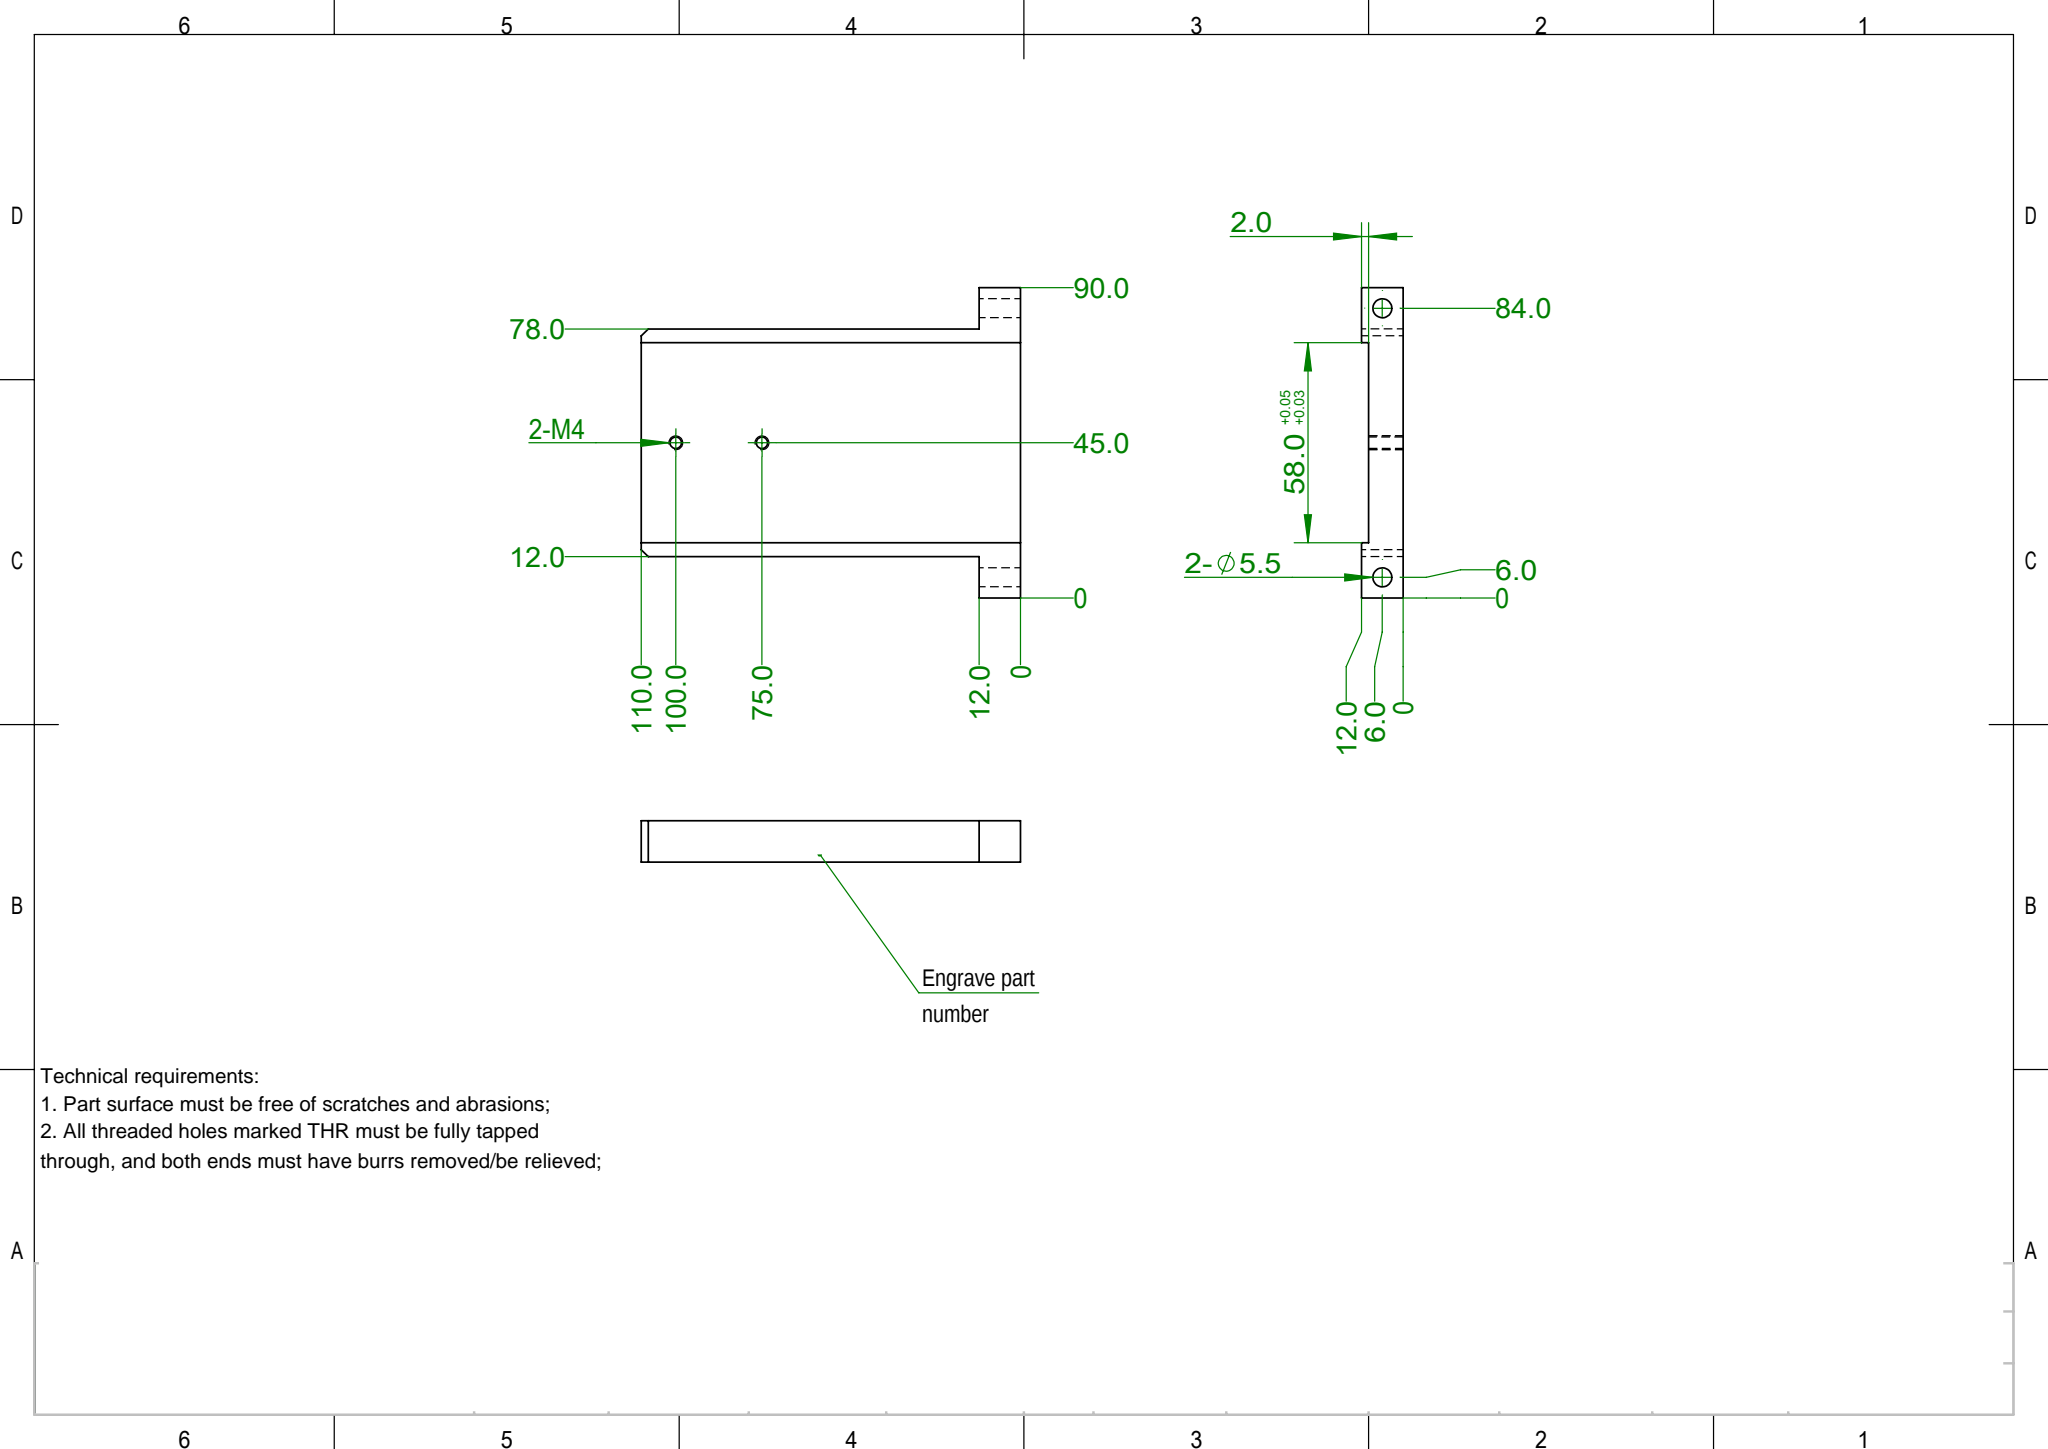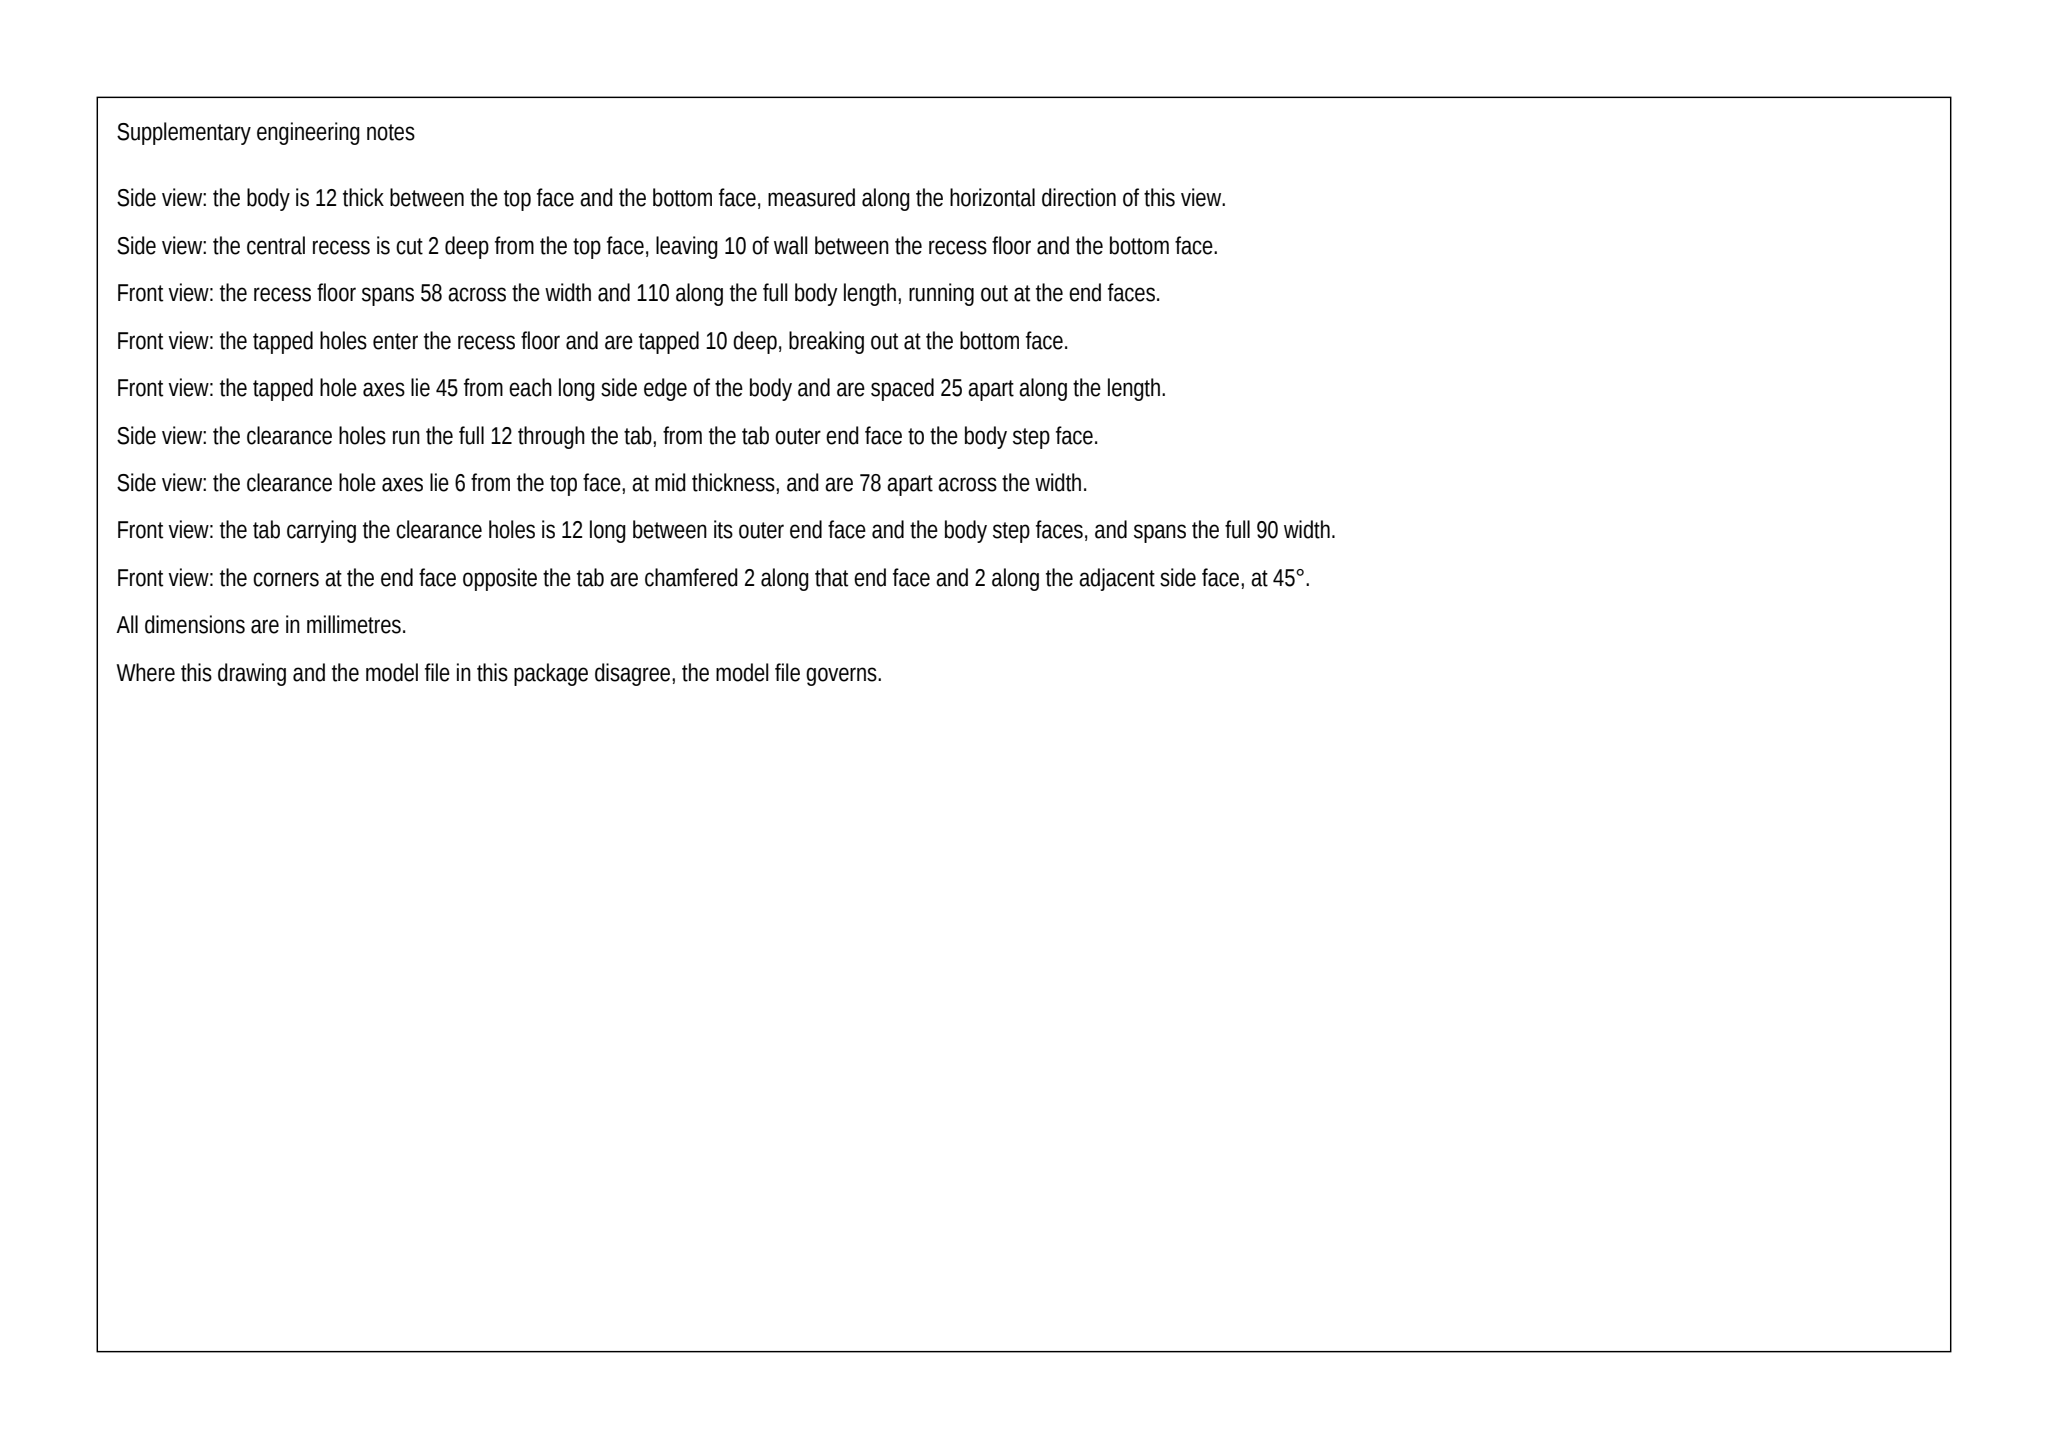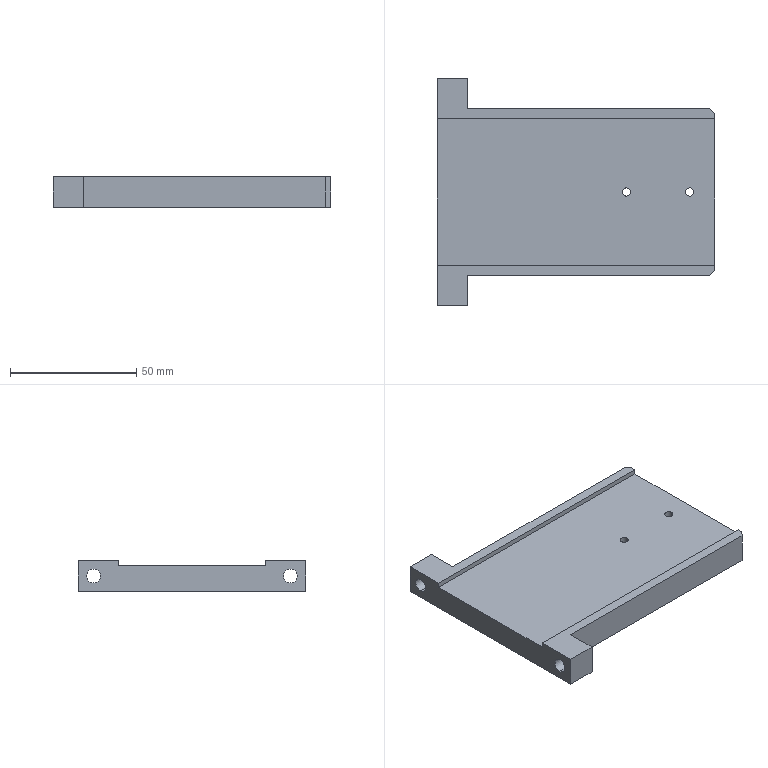Part | SolidWorks | mm | 1 solid | 24 faces | box 110 x 90 x 12 mm | volume 77027 mm3 | plane 16 | cylinder 8 | commonest cylinder face diameters 3.3 x4 5.5 x4
Drawing notes:
FRONT VIEW: 2X C4 ON 110 END CORNERS AT 12.0 & 78.0 | from the solid: y-planes at 16.0 and 74.0 (4 mm in from y=12 and y=78) adjacent to x=110 end face; corner cut 4x4
2.0 DEEP CHANNEL 58.0 WIDE: 16.0 FROM 0 EDGE, SYM ABT 45.0 CL | from the solid: y-planes at 16.0 and 74.0 (58.0 wide) within 0-90 bbox; x-planes 12.0 vs 10.0 give 2.0 depth; midpoint 45.0
2X M4 TAPPED HOLE (Ø3.3 DRILL) 10.0 DEEP, BLIND FROM THE 12.0 TOP FACE (Z=12.0); AT X=75.0 AND X=100.0, Y=45.0 FROM 0 EDGES | from the solid: cylinders [3.3, z, (75.0,45.0), length 10.0] and [3.3, z, (100.0,45.0), length 10.0]; bbox z = 12.0
2.0 DEEP x 58.0 WIDE CHANNEL (Y 16.0 TO 74.0) RUNS FULL LENGTH, X=0 THRU X=110.0; FLOOR AT Z=10.0 | from the solid: axis_planes z=10.0 (channel floor, 1 face) and z=12.0 (top split into 2 faces); single faces at x=0.0 and x=110.0 with bbox x = 110.0; y planes 16.0 and 74.0
build123d program:
from build123d import *

# Parameters (mm, degrees)
SKETCH1_W                  = 105
SKETCH1_H                  = 90
BOSS_EXTRUDE1_DEPTH        = 6
SKETCH2_W                  = 105
SKETCH2_H                  = 58
CUT_EXTRUDE1_DEPTH         = 2
SKETCH3_W                  = 93
SKETCH3_H                  = 12
CUT_EXTRUDE2_DEPTH         = 71.18
F_5_5_5_5_DIAMETER_HOLE1_D = 5.5
M4_TAPPED_HOLE1_D          = 3.3
MOVE_FACE1_BY              = 5
CHAMFER1_SIZE              = 2


with BuildPart() as part:
    # Sketch1 → Boss-Extrude1 (new, symmetric)
    with BuildSketch(Plane.XY):
        Rectangle(SKETCH1_W, SKETCH1_H)
    extrude(amount=BOSS_EXTRUDE1_DEPTH, both=True)

    # Sketch2 → Cut-Extrude1 (cut)
    with BuildSketch(Plane.XY.offset(6)):
        Rectangle(SKETCH2_W, SKETCH2_H)
    extrude(amount=-CUT_EXTRUDE1_DEPTH, mode=Mode.SUBTRACT)

    # Sketch3 → Cut-Extrude2 (cut, through all)
    with BuildSketch(Plane.XY.offset(6)):
        with Locations((6, 39)):
            Rectangle(SKETCH3_W, SKETCH3_H)
        with Locations((6, -39)):
            Rectangle(SKETCH3_W, SKETCH3_H)
    extrude(amount=-CUT_EXTRUDE2_DEPTH, mode=Mode.SUBTRACT)

    # 5.5 _5.5_ Diameter Hole1 (through all)
    with Locations(Plane(origin=(-40.5, 0, 0), x_dir=(0, 0, -1), z_dir=(1, 0, 0))):
        with Locations((0, -39), (0, 39)):
            Hole(F_5_5_5_5_DIAMETER_HOLE1_D / 2)

    # M4 Tapped Hole1 (through all)
    with Locations(Plane.XY.offset(4)):
        with Locations((22.5, 0), (47.5, 0)):
            Hole(M4_TAPPED_HOLE1_D / 2)

    # Move Face1: a face moved outward by 5.0
    extrude(part.faces().sort_by_distance((52.5, 0, -0.858))[0], amount=MOVE_FACE1_BY, dir=(1, 0, 0))

    # Chamfer1
    chamfer1_edges = [part.edges().sort_by_distance(p)[0] for p in [
        (57.5, 33, 0),
        (57.5, -33, 0),
    ]]
    chamfer(chamfer1_edges, length=CHAMFER1_SIZE)


solid = part.part
STEP:
#1=CARTESIAN_POINT('',(20.85,-0.,-6.));
#2=VERTEX_POINT('',#1);
#3=CARTESIAN_POINT('',(24.15,-0.,-6.));
#4=VERTEX_POINT('',#3);
#5=CARTESIAN_POINT('',(22.5,-0.,-6.));
#6=DIRECTION('',(0.,0.,1.));
#7=DIRECTION('',(1.,0.,0.));
#8=AXIS2_PLACEMENT_3D('',#5,#6,#7);
#9=CIRCLE('',#8,1.65);
#10=EDGE_CURVE('',#2,#4,#9,.T.);
#11=ORIENTED_EDGE('',*,*,#10,.F.);
#12=CARTESIAN_POINT('',(20.85,-0.,4.));
#13=VERTEX_POINT('',#12);
#14=CARTESIAN_POINT('',(20.85,-0.,4.));
#15=DIRECTION('',(0.,0.,1.));
#16=VECTOR('',#15,1000.);
#17=LINE('',#14,#16);
#18=EDGE_CURVE('',#2,#13,#17,.T.);
#19=ORIENTED_EDGE('',*,*,#18,.T.);
#20=CARTESIAN_POINT('',(24.15,-0.,4.));
#21=VERTEX_POINT('',#20);
#22=CARTESIAN_POINT('',(22.5,-0.,4.));
#23=DIRECTION('',(0.,0.,1.));
#24=DIRECTION('',(1.,0.,0.));
#25=AXIS2_PLACEMENT_3D('',#22,#23,#24);
#26=CIRCLE('',#25,1.65);
#27=EDGE_CURVE('',#13,#21,#26,.T.);
#28=ORIENTED_EDGE('',*,*,#27,.T.);
#29=CARTESIAN_POINT('',(24.15,-0.,4.));
#30=DIRECTION('',(0.,0.,1.));
#31=VECTOR('',#30,1000.);
#32=LINE('',#29,#31);
#33=EDGE_CURVE('',#4,#21,#32,.T.);
#34=ORIENTED_EDGE('',*,*,#33,.F.);
#35=EDGE_LOOP('',(#11,#19,#28,#34));
#36=FACE_OUTER_BOUND('',#35,.T.);
#37=CARTESIAN_POINT('',(22.5,-0.,4.));
#38=DIRECTION('',(0.,0.,1.));
#39=DIRECTION('',(1.,0.,0.));
#40=AXIS2_PLACEMENT_3D('',#37,#38,#39);
#41=CYLINDRICAL_SURFACE('',#40,1.65);
#42=ADVANCED_FACE('',(#36),#41,.F.);
#43=CARTESIAN_POINT('',(45.85,-0.,-6.));
#44=VERTEX_POINT('',#43);
#45=CARTESIAN_POINT('',(49.15,-0.,-6.));
#46=VERTEX_POINT('',#45);
#47=CARTESIAN_POINT('',(47.5,-0.,-6.));
#48=DIRECTION('',(0.,0.,1.));
#49=DIRECTION('',(1.,0.,0.));
#50=AXIS2_PLACEMENT_3D('',#47,#48,#49);
#51=CIRCLE('',#50,1.65);
#52=EDGE_CURVE('',#44,#46,#51,.T.);
#53=ORIENTED_EDGE('',*,*,#52,.F.);
#54=CARTESIAN_POINT('',(45.85,-0.,4.));
#55=VERTEX_POINT('',#54);
#56=CARTESIAN_POINT('',(45.85,-0.,4.));
#57=DIRECTION('',(0.,0.,1.));
#58=VECTOR('',#57,1000.);
#59=LINE('',#56,#58);
#60=EDGE_CURVE('',#44,#55,#59,.T.);
#61=ORIENTED_EDGE('',*,*,#60,.T.);
#62=CARTESIAN_POINT('',(49.15,-0.,4.));
#63=VERTEX_POINT('',#62);
#64=CARTESIAN_POINT('',(47.5,-0.,4.));
#65=DIRECTION('',(0.,0.,1.));
#66=DIRECTION('',(1.,0.,0.));
#67=AXIS2_PLACEMENT_3D('',#64,#65,#66);
#68=CIRCLE('',#67,1.65);
#69=EDGE_CURVE('',#55,#63,#68,.T.);
#70=ORIENTED_EDGE('',*,*,#69,.T.);
#71=CARTESIAN_POINT('',(49.15,-0.,4.));
#72=DIRECTION('',(0.,0.,1.));
#73=VECTOR('',#72,1000.);
#74=LINE('',#71,#73);
#75=EDGE_CURVE('',#46,#63,#74,.T.);
#76=ORIENTED_EDGE('',*,*,#75,.F.);
#77=EDGE_LOOP('',(#53,#61,#70,#76));
#78=FACE_OUTER_BOUND('',#77,.T.);
#79=CARTESIAN_POINT('',(47.5,-0.,4.));
#80=DIRECTION('',(0.,0.,1.));
#81=DIRECTION('',(1.,0.,0.));
#82=AXIS2_PLACEMENT_3D('',#79,#80,#81);
#83=CYLINDRICAL_SURFACE('',#82,1.65);
#84=ADVANCED_FACE('',(#78),#83,.F.);
#85=CARTESIAN_POINT('',(-52.5,-39.,2.75));
#86=VERTEX_POINT('',#85);
#87=CARTESIAN_POINT('',(-52.5,-39.,-2.75));
#88=VERTEX_POINT('',#87);
#89=CARTESIAN_POINT('',(-52.5,-39.,0.));
#90=DIRECTION('',(1.,0.,0.));
#91=DIRECTION('',(0.,0.,-1.));
#92=AXIS2_PLACEMENT_3D('',#89,#90,#91);
#93=CIRCLE('',#92,2.75);
#94=EDGE_CURVE('',#86,#88,#93,.T.);
#95=ORIENTED_EDGE('',*,*,#94,.F.);
#96=CARTESIAN_POINT('',(-40.5,-39.,2.75));
#97=VERTEX_POINT('',#96);
#98=CARTESIAN_POINT('',(-40.5,-39.,2.75));
#99=DIRECTION('',(1.,0.,0.));
#100=VECTOR('',#99,1000.);
#101=LINE('',#98,#100);
#102=EDGE_CURVE('',#86,#97,#101,.T.);
#103=ORIENTED_EDGE('',*,*,#102,.T.);
#104=CARTESIAN_POINT('',(-40.5,-39.,-2.75));
#105=VERTEX_POINT('',#104);
#106=CARTESIAN_POINT('',(-40.5,-39.,0.));
#107=DIRECTION('',(1.,0.,0.));
#108=DIRECTION('',(0.,0.,-1.));
#109=AXIS2_PLACEMENT_3D('',#106,#107,#108);
#110=CIRCLE('',#109,2.75);
#111=EDGE_CURVE('',#97,#105,#110,.T.);
#112=ORIENTED_EDGE('',*,*,#111,.T.);
#113=CARTESIAN_POINT('',(-40.5,-39.,-2.75));
#114=DIRECTION('',(1.,0.,0.));
#115=VECTOR('',#114,1000.);
#116=LINE('',#113,#115);
#117=EDGE_CURVE('',#88,#105,#116,.T.);
#118=ORIENTED_EDGE('',*,*,#117,.F.);
#119=EDGE_LOOP('',(#95,#103,#112,#118));
#120=FACE_OUTER_BOUND('',#119,.T.);
#121=CARTESIAN_POINT('',(-40.5,-39.,0.));
#122=DIRECTION('',(1.,0.,0.));
#123=DIRECTION('',(0.,0.,-1.));
#124=AXIS2_PLACEMENT_3D('',#121,#122,#123);
#125=CYLINDRICAL_SURFACE('',#124,2.75);
#126=ADVANCED_FACE('',(#120),#125,.F.);
#127=CARTESIAN_POINT('',(-52.5,39.,2.75));
#128=VERTEX_POINT('',#127);
#129=CARTESIAN_POINT('',(-52.5,39.,-2.75));
#130=VERTEX_POINT('',#129);
#131=CARTESIAN_POINT('',(-52.5,39.,0.));
#132=DIRECTION('',(1.,0.,0.));
#133=DIRECTION('',(0.,0.,-1.));
#134=AXIS2_PLACEMENT_3D('',#131,#132,#133);
#135=CIRCLE('',#134,2.75);
#136=EDGE_CURVE('',#128,#130,#135,.T.);
#137=ORIENTED_EDGE('',*,*,#136,.F.);
#138=CARTESIAN_POINT('',(-40.5,39.,2.75));
#139=VERTEX_POINT('',#138);
#140=CARTESIAN_POINT('',(-40.5,39.,2.75));
#141=DIRECTION('',(1.,0.,0.));
#142=VECTOR('',#141,1000.);
#143=LINE('',#140,#142);
#144=EDGE_CURVE('',#128,#139,#143,.T.);
#145=ORIENTED_EDGE('',*,*,#144,.T.);
#146=CARTESIAN_POINT('',(-40.5,39.,-2.75));
#147=VERTEX_POINT('',#146);
#148=CARTESIAN_POINT('',(-40.5,39.,0.));
#149=DIRECTION('',(1.,0.,0.));
#150=DIRECTION('',(0.,0.,-1.));
#151=AXIS2_PLACEMENT_3D('',#148,#149,#150);
#152=CIRCLE('',#151,2.75);
#153=EDGE_CURVE('',#139,#147,#152,.T.);
#154=ORIENTED_EDGE('',*,*,#153,.T.);
#155=CARTESIAN_POINT('',(-40.5,39.,-2.75));
#156=DIRECTION('',(1.,0.,0.));
#157=VECTOR('',#156,1000.);
#158=LINE('',#155,#157);
#159=EDGE_CURVE('',#130,#147,#158,.T.);
#160=ORIENTED_EDGE('',*,*,#159,.F.);
#161=EDGE_LOOP('',(#137,#145,#154,#160));
#162=FACE_OUTER_BOUND('',#161,.T.);
#163=CARTESIAN_POINT('',(-40.5,39.,0.));
#164=DIRECTION('',(1.,0.,0.));
#165=DIRECTION('',(0.,0.,-1.));
#166=AXIS2_PLACEMENT_3D('',#163,#164,#165);
#167=CYLINDRICAL_SURFACE('',#166,2.75);
#168=ADVANCED_FACE('',(#162),#167,.F.);
#169=CARTESIAN_POINT('',(55.5,-33.,6.));
#170=VERTEX_POINT('',#169);
#171=CARTESIAN_POINT('',(-40.5,-33.,6.));
#172=VERTEX_POINT('',#171);
#173=CARTESIAN_POINT('',(52.5,-33.,6.));
#174=DIRECTION('',(-1.,0.,0.));
#175=VECTOR('',#174,1000.);
#176=LINE('',#173,#175);
#177=EDGE_CURVE('',#170,#172,#176,.T.);
#178=ORIENTED_EDGE('',*,*,#177,.F.);
#179=CARTESIAN_POINT('',(57.5,-31.,6.));
#180=VERTEX_POINT('',#179);
#181=CARTESIAN_POINT('',(55.5,-33.,6.));
#182=DIRECTION('',(0.7071,0.7071,0.));
#183=VECTOR('',#182,1000.);
#184=LINE('',#181,#183);
#185=EDGE_CURVE('',#170,#180,#184,.T.);
#186=ORIENTED_EDGE('',*,*,#185,.T.);
#187=CARTESIAN_POINT('',(57.5,-29.,6.));
#188=VERTEX_POINT('',#187);
#189=CARTESIAN_POINT('',(57.5,0.,6.));
#190=DIRECTION('',(0.,1.,0.));
#191=VECTOR('',#190,1000.);
#192=LINE('',#189,#191);
#193=EDGE_CURVE('',#180,#188,#192,.T.);
#194=ORIENTED_EDGE('',*,*,#193,.T.);
#195=CARTESIAN_POINT('',(-52.5,-29.,6.));
#196=VERTEX_POINT('',#195);
#197=CARTESIAN_POINT('',(-52.5,-29.,6.));
#198=DIRECTION('',(1.,0.,0.));
#199=VECTOR('',#198,1000.);
#200=LINE('',#197,#199);
#201=EDGE_CURVE('',#196,#188,#200,.T.);
#202=ORIENTED_EDGE('',*,*,#201,.F.);
#203=CARTESIAN_POINT('',(-52.5,-45.,6.));
#204=VERTEX_POINT('',#203);
#205=CARTESIAN_POINT('',(-52.5,-45.,6.));
#206=DIRECTION('',(0.,-1.,0.));
#207=VECTOR('',#206,1000.);
#208=LINE('',#205,#207);
#209=EDGE_CURVE('',#196,#204,#208,.T.);
#210=ORIENTED_EDGE('',*,*,#209,.T.);
#211=CARTESIAN_POINT('',(-40.5,-45.,6.));
#212=VERTEX_POINT('',#211);
#213=CARTESIAN_POINT('',(-52.5,-45.,6.));
#214=DIRECTION('',(1.,0.,0.));
#215=VECTOR('',#214,1000.);
#216=LINE('',#213,#215);
#217=EDGE_CURVE('',#204,#212,#216,.T.);
#218=ORIENTED_EDGE('',*,*,#217,.T.);
#219=CARTESIAN_POINT('',(-40.5,-45.,6.));
#220=DIRECTION('',(0.,-1.,0.));
#221=VECTOR('',#220,1000.);
#222=LINE('',#219,#221);
#223=EDGE_CURVE('',#172,#212,#222,.T.);
#224=ORIENTED_EDGE('',*,*,#223,.F.);
#225=EDGE_LOOP('',(#178,#186,#194,#202,#210,#218,#224));
#226=FACE_OUTER_BOUND('',#225,.T.);
#227=CARTESIAN_POINT('',(0.,0.,6.));
#228=DIRECTION('',(0.,0.,-1.));
#229=DIRECTION('',(-1.,0.,0.));
#230=AXIS2_PLACEMENT_3D('',#227,#228,#229);
#231=PLANE('',#230);
#232=ADVANCED_FACE('',(#226),#231,.F.);
#233=ORIENTED_EDGE('',*,*,#193,.F.);
#234=CARTESIAN_POINT('',(57.5,-31.,-6.));
#235=VERTEX_POINT('',#234);
#236=CARTESIAN_POINT('',(57.5,-31.,6.));
#237=DIRECTION('',(0.,0.,-1.));
#238=VECTOR('',#237,1000.);
#239=LINE('',#236,#238);
#240=EDGE_CURVE('',#180,#235,#239,.T.);
#241=ORIENTED_EDGE('',*,*,#240,.T.);
#242=CARTESIAN_POINT('',(57.5,31.,-6.));
#243=VERTEX_POINT('',#242);
#244=CARTESIAN_POINT('',(57.5,0.,-6.));
#245=DIRECTION('',(0.,1.,0.));
#246=VECTOR('',#245,1000.);
#247=LINE('',#244,#246);
#248=EDGE_CURVE('',#235,#243,#247,.T.);
#249=ORIENTED_EDGE('',*,*,#248,.T.);
#250=CARTESIAN_POINT('',(57.5,31.,6.));
#251=VERTEX_POINT('',#250);
#252=CARTESIAN_POINT('',(57.5,31.,6.));
#253=DIRECTION('',(0.,0.,1.));
#254=VECTOR('',#253,1000.);
#255=LINE('',#252,#254);
#256=EDGE_CURVE('',#243,#251,#255,.T.);
#257=ORIENTED_EDGE('',*,*,#256,.T.);
#258=CARTESIAN_POINT('',(57.5,29.,6.));
#259=VERTEX_POINT('',#258);
#260=CARTESIAN_POINT('',(57.5,0.,6.));
#261=DIRECTION('',(0.,1.,0.));
#262=VECTOR('',#261,1000.);
#263=LINE('',#260,#262);
#264=EDGE_CURVE('',#259,#251,#263,.T.);
#265=ORIENTED_EDGE('',*,*,#264,.F.);
#266=CARTESIAN_POINT('',(57.5,29.,4.));
#267=VERTEX_POINT('',#266);
#268=CARTESIAN_POINT('',(57.5,29.,4.));
#269=DIRECTION('',(0.,0.,1.));
#270=VECTOR('',#269,1000.);
#271=LINE('',#268,#270);
#272=EDGE_CURVE('',#267,#259,#271,.T.);
#273=ORIENTED_EDGE('',*,*,#272,.F.);
#274=CARTESIAN_POINT('',(57.5,-29.,4.));
#275=VERTEX_POINT('',#274);
#276=CARTESIAN_POINT('',(57.5,0.,4.));
#277=DIRECTION('',(0.,1.,0.));
#278=VECTOR('',#277,1000.);
#279=LINE('',#276,#278);
#280=EDGE_CURVE('',#275,#267,#279,.T.);
#281=ORIENTED_EDGE('',*,*,#280,.F.);
#282=CARTESIAN_POINT('',(57.5,-29.,6.));
#283=DIRECTION('',(0.,0.,1.));
#284=VECTOR('',#283,1000.);
#285=LINE('',#282,#284);
#286=EDGE_CURVE('',#275,#188,#285,.T.);
#287=ORIENTED_EDGE('',*,*,#286,.T.);
#288=EDGE_LOOP('',(#233,#241,#249,#257,#265,#273,#281,#287));
#289=FACE_OUTER_BOUND('',#288,.T.);
#290=CARTESIAN_POINT('',(57.5,-45.,6.));
#291=DIRECTION('',(-1.,0.,0.));
#292=DIRECTION('',(0.,0.,1.));
#293=AXIS2_PLACEMENT_3D('',#290,#291,#292);
#294=PLANE('',#293);
#295=ADVANCED_FACE('',(#289),#294,.F.);
#296=CARTESIAN_POINT('',(-40.5,45.,6.));
#297=VERTEX_POINT('',#296);
#298=CARTESIAN_POINT('',(-52.5,45.,6.));
#299=VERTEX_POINT('',#298);
#300=CARTESIAN_POINT('',(-52.5,45.,6.));
#301=DIRECTION('',(-1.,0.,0.));
#302=VECTOR('',#301,1000.);
#303=LINE('',#300,#302);
#304=EDGE_CURVE('',#297,#299,#303,.T.);
#305=ORIENTED_EDGE('',*,*,#304,.F.);
#306=CARTESIAN_POINT('',(-40.5,45.,-6.));
#307=VERTEX_POINT('',#306);
#308=CARTESIAN_POINT('',(-40.5,45.,-6.));
#309=DIRECTION('',(0.,0.,1.));
#310=VECTOR('',#309,1000.);
#311=LINE('',#308,#310);
#312=EDGE_CURVE('',#307,#297,#311,.T.);
#313=ORIENTED_EDGE('',*,*,#312,.F.);
#314=CARTESIAN_POINT('',(-52.5,45.,-6.));
#315=VERTEX_POINT('',#314);
#316=CARTESIAN_POINT('',(-52.5,45.,-6.));
#317=DIRECTION('',(-1.,0.,0.));
#318=VECTOR('',#317,1000.);
#319=LINE('',#316,#318);
#320=EDGE_CURVE('',#307,#315,#319,.T.);
#321=ORIENTED_EDGE('',*,*,#320,.T.);
#322=CARTESIAN_POINT('',(-52.5,45.,6.));
#323=DIRECTION('',(0.,0.,-1.));
#324=VECTOR('',#323,1000.);
#325=LINE('',#322,#324);
#326=EDGE_CURVE('',#299,#315,#325,.T.);
#327=ORIENTED_EDGE('',*,*,#326,.F.);
#328=EDGE_LOOP('',(#305,#313,#321,#327));
#329=FACE_OUTER_BOUND('',#328,.T.);
#330=CARTESIAN_POINT('',(-52.5,45.,6.));
#331=DIRECTION('',(0.,-1.,0.));
#332=DIRECTION('',(0.,0.,-1.));
#333=AXIS2_PLACEMENT_3D('',#330,#331,#332);
#334=PLANE('',#333);
#335=ADVANCED_FACE('',(#329),#334,.F.);
#336=CARTESIAN_POINT('',(-52.5,-39.,0.));
#337=DIRECTION('',(1.,0.,0.));
#338=DIRECTION('',(0.,0.,-1.));
#339=AXIS2_PLACEMENT_3D('',#336,#337,#338);
#340=CIRCLE('',#339,2.75);
#341=EDGE_CURVE('',#88,#86,#340,.T.);
#342=ORIENTED_EDGE('',*,*,#341,.T.);
#343=ORIENTED_EDGE('',*,*,#94,.T.);
#344=EDGE_LOOP('',(#342,#343));
#345=FACE_BOUND('',#344,.T.);
#346=CARTESIAN_POINT('',(-52.5,39.,0.));
#347=DIRECTION('',(1.,0.,0.));
#348=DIRECTION('',(0.,0.,-1.));
#349=AXIS2_PLACEMENT_3D('',#346,#347,#348);
#350=CIRCLE('',#349,2.75);
#351=EDGE_CURVE('',#130,#128,#350,.T.);
#352=ORIENTED_EDGE('',*,*,#351,.T.);
#353=ORIENTED_EDGE('',*,*,#136,.T.);
#354=EDGE_LOOP('',(#352,#353));
#355=FACE_BOUND('',#354,.T.);
#356=ORIENTED_EDGE('',*,*,#209,.F.);
#357=CARTESIAN_POINT('',(-52.5,-29.,4.));
#358=VERTEX_POINT('',#357);
#359=CARTESIAN_POINT('',(-52.5,-29.,4.));
#360=DIRECTION('',(0.,0.,1.));
#361=VECTOR('',#360,1000.);
#362=LINE('',#359,#361);
#363=EDGE_CURVE('',#358,#196,#362,.T.);
#364=ORIENTED_EDGE('',*,*,#363,.F.);
#365=CARTESIAN_POINT('',(-52.5,29.,4.));
#366=VERTEX_POINT('',#365);
#367=CARTESIAN_POINT('',(-52.5,-29.,4.));
#368=DIRECTION('',(0.,-1.,0.));
#369=VECTOR('',#368,1000.);
#370=LINE('',#367,#369);
#371=EDGE_CURVE('',#366,#358,#370,.T.);
#372=ORIENTED_EDGE('',*,*,#371,.F.);
#373=CARTESIAN_POINT('',(-52.5,29.,6.));
#374=VERTEX_POINT('',#373);
#375=CARTESIAN_POINT('',(-52.5,29.,4.));
#376=DIRECTION('',(0.,0.,1.));
#377=VECTOR('',#376,1000.);
#378=LINE('',#375,#377);
#379=EDGE_CURVE('',#366,#374,#378,.T.);
#380=ORIENTED_EDGE('',*,*,#379,.T.);
#381=CARTESIAN_POINT('',(-52.5,-45.,6.));
#382=DIRECTION('',(0.,-1.,0.));
#383=VECTOR('',#382,1000.);
#384=LINE('',#381,#383);
#385=EDGE_CURVE('',#299,#374,#384,.T.);
#386=ORIENTED_EDGE('',*,*,#385,.F.);
#387=ORIENTED_EDGE('',*,*,#326,.T.);
#388=CARTESIAN_POINT('',(-52.5,-45.,-6.));
#389=VERTEX_POINT('',#388);
#390=CARTESIAN_POINT('',(-52.5,-45.,-6.));
#391=DIRECTION('',(0.,-1.,0.));
#392=VECTOR('',#391,1000.);
#393=LINE('',#390,#392);
#394=EDGE_CURVE('',#315,#389,#393,.T.);
#395=ORIENTED_EDGE('',*,*,#394,.T.);
#396=CARTESIAN_POINT('',(-52.5,-45.,6.));
#397=DIRECTION('',(0.,0.,-1.));
#398=VECTOR('',#397,1000.);
#399=LINE('',#396,#398);
#400=EDGE_CURVE('',#204,#389,#399,.T.);
#401=ORIENTED_EDGE('',*,*,#400,.F.);
#402=EDGE_LOOP('',(#356,#364,#372,#380,#386,#387,#395,#401));
#403=FACE_OUTER_BOUND('',#402,.T.);
#404=CARTESIAN_POINT('',(-52.5,-45.,6.));
#405=DIRECTION('',(1.,0.,0.));
#406=DIRECTION('',(0.,0.,-1.));
#407=AXIS2_PLACEMENT_3D('',#404,#405,#406);
#408=PLANE('',#407);
#409=ADVANCED_FACE('',(#345,#355,#403),#408,.F.);
#410=CARTESIAN_POINT('',(-40.5,-45.,-6.));
#411=VERTEX_POINT('',#410);
#412=CARTESIAN_POINT('',(-52.5,-45.,-6.));
#413=DIRECTION('',(1.,0.,0.));
#414=VECTOR('',#413,1000.);
#415=LINE('',#412,#414);
#416=EDGE_CURVE('',#389,#411,#415,.T.);
#417=ORIENTED_EDGE('',*,*,#416,.T.);
#418=CARTESIAN_POINT('',(-40.5,-45.,-6.));
#419=DIRECTION('',(0.,0.,1.));
#420=VECTOR('',#419,1000.);
#421=LINE('',#418,#420);
#422=EDGE_CURVE('',#411,#212,#421,.T.);
#423=ORIENTED_EDGE('',*,*,#422,.T.);
#424=ORIENTED_EDGE('',*,*,#217,.F.);
#425=ORIENTED_EDGE('',*,*,#400,.T.);
#426=EDGE_LOOP('',(#417,#423,#424,#425));
#427=FACE_OUTER_BOUND('',#426,.T.);
#428=CARTESIAN_POINT('',(-52.5,-45.,6.));
#429=DIRECTION('',(0.,1.,0.));
#430=DIRECTION('',(0.,0.,1.));
#431=AXIS2_PLACEMENT_3D('',#428,#429,#430);
#432=PLANE('',#431);
#433=ADVANCED_FACE('',(#427),#432,.F.);
#434=ORIENTED_EDGE('',*,*,#264,.T.);
#435=CARTESIAN_POINT('',(55.5,33.,6.));
#436=VERTEX_POINT('',#435);
#437=CARTESIAN_POINT('',(57.5,31.,6.));
#438=DIRECTION('',(-0.7071,0.7071,0.));
#439=VECTOR('',#438,1000.);
#440=LINE('',#437,#439);
#441=EDGE_CURVE('',#251,#436,#440,.T.);
#442=ORIENTED_EDGE('',*,*,#441,.T.);
#443=CARTESIAN_POINT('',(-40.5,33.,6.));
#444=VERTEX_POINT('',#443);
#445=CARTESIAN_POINT('',(52.5,33.,6.));
#446=DIRECTION('',(1.,0.,0.));
#447=VECTOR('',#446,1000.);
#448=LINE('',#445,#447);
#449=EDGE_CURVE('',#444,#436,#448,.T.);
#450=ORIENTED_EDGE('',*,*,#449,.F.);
#451=CARTESIAN_POINT('',(-40.5,45.,6.));
#452=DIRECTION('',(0.,-1.,0.));
#453=VECTOR('',#452,1000.);
#454=LINE('',#451,#453);
#455=EDGE_CURVE('',#297,#444,#454,.T.);
#456=ORIENTED_EDGE('',*,*,#455,.F.);
#457=ORIENTED_EDGE('',*,*,#304,.T.);
#458=ORIENTED_EDGE('',*,*,#385,.T.);
#459=CARTESIAN_POINT('',(-52.5,29.,6.));
#460=DIRECTION('',(-1.,0.,0.));
#461=VECTOR('',#460,1000.);
#462=LINE('',#459,#461);
#463=EDGE_CURVE('',#259,#374,#462,.T.);
#464=ORIENTED_EDGE('',*,*,#463,.F.);
#465=EDGE_LOOP('',(#434,#442,#450,#456,#457,#458,#464));
#466=FACE_OUTER_BOUND('',#465,.T.);
#467=CARTESIAN_POINT('',(0.,0.,6.));
#468=DIRECTION('',(0.,0.,-1.));
#469=DIRECTION('',(-1.,0.,0.));
#470=AXIS2_PLACEMENT_3D('',#467,#468,#469);
#471=PLANE('',#470);
#472=ADVANCED_FACE('',(#466),#471,.F.);
#473=CARTESIAN_POINT('',(22.5,-0.,-6.));
#474=DIRECTION('',(0.,0.,1.));
#475=DIRECTION('',(1.,0.,0.));
#476=AXIS2_PLACEMENT_3D('',#473,#474,#475);
#477=CIRCLE('',#476,1.65);
#478=EDGE_CURVE('',#4,#2,#477,.T.);
#479=ORIENTED_EDGE('',*,*,#478,.T.);
#480=ORIENTED_EDGE('',*,*,#10,.T.);
#481=EDGE_LOOP('',(#479,#480));
#482=FACE_BOUND('',#481,.T.);
#483=CARTESIAN_POINT('',(47.5,-0.,-6.));
#484=DIRECTION('',(0.,0.,1.));
#485=DIRECTION('',(1.,0.,0.));
#486=AXIS2_PLACEMENT_3D('',#483,#484,#485);
#487=CIRCLE('',#486,1.65);
#488=EDGE_CURVE('',#46,#44,#487,.T.);
#489=ORIENTED_EDGE('',*,*,#488,.T.);
#490=ORIENTED_EDGE('',*,*,#52,.T.);
#491=EDGE_LOOP('',(#489,#490));
#492=FACE_BOUND('',#491,.T.);
#493=ORIENTED_EDGE('',*,*,#248,.F.);
#494=CARTESIAN_POINT('',(55.5,-33.,-6.));
#495=VERTEX_POINT('',#494);
#496=CARTESIAN_POINT('',(44.25,-44.25,-6.));
#497=DIRECTION('',(-0.7071,-0.7071,0.));
#498=VECTOR('',#497,1000.);
#499=LINE('',#496,#498);
#500=EDGE_CURVE('',#235,#495,#499,.T.);
#501=ORIENTED_EDGE('',*,*,#500,.T.);
#502=CARTESIAN_POINT('',(-40.5,-33.,-6.));
#503=VERTEX_POINT('',#502);
#504=CARTESIAN_POINT('',(52.5,-33.,-6.));
#505=DIRECTION('',(-1.,0.,0.));
#506=VECTOR('',#505,1000.);
#507=LINE('',#504,#506);
#508=EDGE_CURVE('',#495,#503,#507,.T.);
#509=ORIENTED_EDGE('',*,*,#508,.T.);
#510=CARTESIAN_POINT('',(-40.5,-45.,-6.));
#511=DIRECTION('',(0.,-1.,0.));
#512=VECTOR('',#511,1000.);
#513=LINE('',#510,#512);
#514=EDGE_CURVE('',#503,#411,#513,.T.);
#515=ORIENTED_EDGE('',*,*,#514,.T.);
#516=ORIENTED_EDGE('',*,*,#416,.F.);
#517=ORIENTED_EDGE('',*,*,#394,.F.);
#518=ORIENTED_EDGE('',*,*,#320,.F.);
#519=CARTESIAN_POINT('',(-40.5,33.,-6.));
#520=VERTEX_POINT('',#519);
#521=CARTESIAN_POINT('',(-40.5,45.,-6.));
#522=DIRECTION('',(0.,-1.,0.));
#523=VECTOR('',#522,1000.);
#524=LINE('',#521,#523);
#525=EDGE_CURVE('',#307,#520,#524,.T.);
#526=ORIENTED_EDGE('',*,*,#525,.T.);
#527=CARTESIAN_POINT('',(55.5,33.,-6.));
#528=VERTEX_POINT('',#527);
#529=CARTESIAN_POINT('',(52.5,33.,-6.));
#530=DIRECTION('',(1.,0.,0.));
#531=VECTOR('',#530,1000.);
#532=LINE('',#529,#531);
#533=EDGE_CURVE('',#520,#528,#532,.T.);
#534=ORIENTED_EDGE('',*,*,#533,.T.);
#535=CARTESIAN_POINT('',(44.25,44.25,-6.));
#536=DIRECTION('',(0.7071,-0.7071,0.));
#537=VECTOR('',#536,1000.);
#538=LINE('',#535,#537);
#539=EDGE_CURVE('',#528,#243,#538,.T.);
#540=ORIENTED_EDGE('',*,*,#539,.T.);
#541=EDGE_LOOP('',(#493,#501,#509,#515,#516,#517,#518,#526,#534,#540));
#542=FACE_OUTER_BOUND('',#541,.T.);
#543=CARTESIAN_POINT('',(0.,0.,-6.));
#544=DIRECTION('',(0.,0.,-1.));
#545=DIRECTION('',(-1.,0.,0.));
#546=AXIS2_PLACEMENT_3D('',#543,#544,#545);
#547=PLANE('',#546);
#548=ADVANCED_FACE('',(#482,#492,#542),#547,.T.);
#549=ORIENTED_EDGE('',*,*,#201,.T.);
#550=ORIENTED_EDGE('',*,*,#286,.F.);
#551=CARTESIAN_POINT('',(-52.5,-29.,4.));
#552=DIRECTION('',(1.,0.,0.));
#553=VECTOR('',#552,1000.);
#554=LINE('',#551,#553);
#555=EDGE_CURVE('',#358,#275,#554,.T.);
#556=ORIENTED_EDGE('',*,*,#555,.F.);
#557=ORIENTED_EDGE('',*,*,#363,.T.);
#558=EDGE_LOOP('',(#549,#550,#556,#557));
#559=FACE_OUTER_BOUND('',#558,.T.);
#560=CARTESIAN_POINT('',(-52.5,-29.,4.));
#561=DIRECTION('',(0.,-1.,0.));
#562=DIRECTION('',(0.,0.,-1.));
#563=AXIS2_PLACEMENT_3D('',#560,#561,#562);
#564=PLANE('',#563);
#565=ADVANCED_FACE('',(#559),#564,.F.);
#566=ORIENTED_EDGE('',*,*,#463,.T.);
#567=ORIENTED_EDGE('',*,*,#379,.F.);
#568=CARTESIAN_POINT('',(-52.5,29.,4.));
#569=DIRECTION('',(-1.,0.,0.));
#570=VECTOR('',#569,1000.);
#571=LINE('',#568,#570);
#572=EDGE_CURVE('',#267,#366,#571,.T.);
#573=ORIENTED_EDGE('',*,*,#572,.F.);
#574=ORIENTED_EDGE('',*,*,#272,.T.);
#575=EDGE_LOOP('',(#566,#567,#573,#574));
#576=FACE_OUTER_BOUND('',#575,.T.);
#577=CARTESIAN_POINT('',(-52.5,29.,4.));
#578=DIRECTION('',(0.,1.,0.));
#579=DIRECTION('',(0.,0.,1.));
#580=AXIS2_PLACEMENT_3D('',#577,#578,#579);
#581=PLANE('',#580);
#582=ADVANCED_FACE('',(#576),#581,.F.);
#583=CARTESIAN_POINT('',(22.5,-0.,4.));
#584=DIRECTION('',(0.,0.,1.));
#585=DIRECTION('',(1.,0.,0.));
#586=AXIS2_PLACEMENT_3D('',#583,#584,#585);
#587=CIRCLE('',#586,1.65);
#588=EDGE_CURVE('',#21,#13,#587,.T.);
#589=ORIENTED_EDGE('',*,*,#588,.F.);
#590=ORIENTED_EDGE('',*,*,#27,.F.);
#591=EDGE_LOOP('',(#589,#590));
#592=FACE_BOUND('',#591,.T.);
#593=CARTESIAN_POINT('',(47.5,-0.,4.));
#594=DIRECTION('',(0.,0.,1.));
#595=DIRECTION('',(1.,0.,0.));
#596=AXIS2_PLACEMENT_3D('',#593,#594,#595);
#597=CIRCLE('',#596,1.65);
#598=EDGE_CURVE('',#63,#55,#597,.T.);
#599=ORIENTED_EDGE('',*,*,#598,.F.);
#600=ORIENTED_EDGE('',*,*,#69,.F.);
#601=EDGE_LOOP('',(#599,#600));
#602=FACE_BOUND('',#601,.T.);
#603=ORIENTED_EDGE('',*,*,#280,.T.);
#604=ORIENTED_EDGE('',*,*,#572,.T.);
#605=ORIENTED_EDGE('',*,*,#371,.T.);
#606=ORIENTED_EDGE('',*,*,#555,.T.);
#607=EDGE_LOOP('',(#603,#604,#605,#606));
#608=FACE_OUTER_BOUND('',#607,.T.);
#609=CARTESIAN_POINT('',(0.,0.,4.));
#610=DIRECTION('',(0.,0.,-1.));
#611=DIRECTION('',(-1.,0.,0.));
#612=AXIS2_PLACEMENT_3D('',#609,#610,#611);
#613=PLANE('',#612);
#614=ADVANCED_FACE('',(#592,#602,#608),#613,.F.);
#615=ORIENTED_EDGE('',*,*,#449,.T.);
#616=CARTESIAN_POINT('',(55.5,33.,-6.));
#617=DIRECTION('',(0.,0.,-1.));
#618=VECTOR('',#617,1000.);
#619=LINE('',#616,#618);
#620=EDGE_CURVE('',#436,#528,#619,.T.);
#621=ORIENTED_EDGE('',*,*,#620,.T.);
#622=ORIENTED_EDGE('',*,*,#533,.F.);
#623=CARTESIAN_POINT('',(-40.5,33.,-6.));
#624=DIRECTION('',(0.,0.,1.));
#625=VECTOR('',#624,1000.);
#626=LINE('',#623,#625);
#627=EDGE_CURVE('',#520,#444,#626,.T.);
#628=ORIENTED_EDGE('',*,*,#627,.T.);
#629=EDGE_LOOP('',(#615,#621,#622,#628));
#630=FACE_OUTER_BOUND('',#629,.T.);
#631=CARTESIAN_POINT('',(52.5,33.,-6.));
#632=DIRECTION('',(0.,-1.,0.));
#633=DIRECTION('',(1.,0.,0.));
#634=AXIS2_PLACEMENT_3D('',#631,#632,#633);
#635=PLANE('',#634);
#636=ADVANCED_FACE('',(#630),#635,.F.);
#637=CARTESIAN_POINT('',(-40.5,39.,0.));
#638=DIRECTION('',(1.,0.,0.));
#639=DIRECTION('',(0.,0.,-1.));
#640=AXIS2_PLACEMENT_3D('',#637,#638,#639);
#641=CIRCLE('',#640,2.75);
#642=EDGE_CURVE('',#147,#139,#641,.T.);
#643=ORIENTED_EDGE('',*,*,#642,.F.);
#644=ORIENTED_EDGE('',*,*,#153,.F.);
#645=EDGE_LOOP('',(#643,#644));
#646=FACE_BOUND('',#645,.T.);
#647=ORIENTED_EDGE('',*,*,#455,.T.);
#648=ORIENTED_EDGE('',*,*,#627,.F.);
#649=ORIENTED_EDGE('',*,*,#525,.F.);
#650=ORIENTED_EDGE('',*,*,#312,.T.);
#651=EDGE_LOOP('',(#647,#648,#649,#650));
#652=FACE_OUTER_BOUND('',#651,.T.);
#653=CARTESIAN_POINT('',(-40.5,45.,-6.));
#654=DIRECTION('',(-1.,0.,0.));
#655=DIRECTION('',(0.,0.,1.));
#656=AXIS2_PLACEMENT_3D('',#653,#654,#655);
#657=PLANE('',#656);
#658=ADVANCED_FACE('',(#646,#652),#657,.F.);
#659=CARTESIAN_POINT('',(-40.5,-39.,0.));
#660=DIRECTION('',(1.,0.,0.));
#661=DIRECTION('',(0.,0.,-1.));
#662=AXIS2_PLACEMENT_3D('',#659,#660,#661);
#663=CIRCLE('',#662,2.75);
#664=EDGE_CURVE('',#105,#97,#663,.T.);
#665=ORIENTED_EDGE('',*,*,#664,.F.);
#666=ORIENTED_EDGE('',*,*,#111,.F.);
#667=EDGE_LOOP('',(#665,#666));
#668=FACE_BOUND('',#667,.T.);
#669=ORIENTED_EDGE('',*,*,#223,.T.);
#670=ORIENTED_EDGE('',*,*,#422,.F.);
#671=ORIENTED_EDGE('',*,*,#514,.F.);
#672=CARTESIAN_POINT('',(-40.5,-33.,-6.));
#673=DIRECTION('',(0.,0.,1.));
#674=VECTOR('',#673,1000.);
#675=LINE('',#672,#674);
#676=EDGE_CURVE('',#503,#172,#675,.T.);
#677=ORIENTED_EDGE('',*,*,#676,.T.);
#678=EDGE_LOOP('',(#669,#670,#671,#677));
#679=FACE_OUTER_BOUND('',#678,.T.);
#680=CARTESIAN_POINT('',(-40.5,-45.,-6.));
#681=DIRECTION('',(-1.,0.,0.));
#682=DIRECTION('',(0.,0.,1.));
#683=AXIS2_PLACEMENT_3D('',#680,#681,#682);
#684=PLANE('',#683);
#685=ADVANCED_FACE('',(#668,#679),#684,.F.);
#686=ORIENTED_EDGE('',*,*,#508,.F.);
#687=CARTESIAN_POINT('',(55.5,-33.,-6.));
#688=DIRECTION('',(0.,0.,1.));
#689=VECTOR('',#688,1000.);
#690=LINE('',#687,#689);
#691=EDGE_CURVE('',#495,#170,#690,.T.);
#692=ORIENTED_EDGE('',*,*,#691,.T.);
#693=ORIENTED_EDGE('',*,*,#177,.T.);
#694=ORIENTED_EDGE('',*,*,#676,.F.);
#695=EDGE_LOOP('',(#686,#692,#693,#694));
#696=FACE_OUTER_BOUND('',#695,.T.);
#697=CARTESIAN_POINT('',(52.5,-33.,-6.));
#698=DIRECTION('',(0.,1.,0.));
#699=DIRECTION('',(-1.,0.,0.));
#700=AXIS2_PLACEMENT_3D('',#697,#698,#699);
#701=PLANE('',#700);
#702=ADVANCED_FACE('',(#696),#701,.F.);
#703=ORIENTED_EDGE('',*,*,#144,.F.);
#704=ORIENTED_EDGE('',*,*,#351,.F.);
#705=ORIENTED_EDGE('',*,*,#159,.T.);
#706=ORIENTED_EDGE('',*,*,#642,.T.);
#707=EDGE_LOOP('',(#703,#704,#705,#706));
#708=FACE_OUTER_BOUND('',#707,.T.);
#709=CARTESIAN_POINT('',(-40.5,39.,0.));
#710=DIRECTION('',(1.,0.,0.));
#711=DIRECTION('',(0.,0.,-1.));
#712=AXIS2_PLACEMENT_3D('',#709,#710,#711);
#713=CYLINDRICAL_SURFACE('',#712,2.75);
#714=ADVANCED_FACE('',(#708),#713,.F.);
#715=ORIENTED_EDGE('',*,*,#102,.F.);
#716=ORIENTED_EDGE('',*,*,#341,.F.);
#717=ORIENTED_EDGE('',*,*,#117,.T.);
#718=ORIENTED_EDGE('',*,*,#664,.T.);
#719=EDGE_LOOP('',(#715,#716,#717,#718));
#720=FACE_OUTER_BOUND('',#719,.T.);
#721=CARTESIAN_POINT('',(-40.5,-39.,0.));
#722=DIRECTION('',(1.,0.,0.));
#723=DIRECTION('',(0.,0.,-1.));
#724=AXIS2_PLACEMENT_3D('',#721,#722,#723);
#725=CYLINDRICAL_SURFACE('',#724,2.75);
#726=ADVANCED_FACE('',(#720),#725,.F.);
#727=ORIENTED_EDGE('',*,*,#60,.F.);
#728=ORIENTED_EDGE('',*,*,#488,.F.);
#729=ORIENTED_EDGE('',*,*,#75,.T.);
#730=ORIENTED_EDGE('',*,*,#598,.T.);
#731=EDGE_LOOP('',(#727,#728,#729,#730));
#732=FACE_OUTER_BOUND('',#731,.T.);
#733=CARTESIAN_POINT('',(47.5,-0.,4.));
#734=DIRECTION('',(0.,0.,1.));
#735=DIRECTION('',(1.,0.,0.));
#736=AXIS2_PLACEMENT_3D('',#733,#734,#735);
#737=CYLINDRICAL_SURFACE('',#736,1.65);
#738=ADVANCED_FACE('',(#732),#737,.F.);
#739=ORIENTED_EDGE('',*,*,#18,.F.);
#740=ORIENTED_EDGE('',*,*,#478,.F.);
#741=ORIENTED_EDGE('',*,*,#33,.T.);
#742=ORIENTED_EDGE('',*,*,#588,.T.);
#743=EDGE_LOOP('',(#739,#740,#741,#742));
#744=FACE_OUTER_BOUND('',#743,.T.);
#745=CARTESIAN_POINT('',(22.5,-0.,4.));
#746=DIRECTION('',(0.,0.,1.));
#747=DIRECTION('',(1.,0.,0.));
#748=AXIS2_PLACEMENT_3D('',#745,#746,#747);
#749=CYLINDRICAL_SURFACE('',#748,1.65);
#750=ADVANCED_FACE('',(#744),#749,.F.);
#751=ORIENTED_EDGE('',*,*,#500,.F.);
#752=ORIENTED_EDGE('',*,*,#240,.F.);
#753=ORIENTED_EDGE('',*,*,#185,.F.);
#754=ORIENTED_EDGE('',*,*,#691,.F.);
#755=EDGE_LOOP('',(#751,#752,#753,#754));
#756=FACE_OUTER_BOUND('',#755,.T.);
#757=CARTESIAN_POINT('',(55.5,-33.,-6.));
#758=DIRECTION('',(-0.7071,0.7071,0.));
#759=DIRECTION('',(0.,0.,1.));
#760=AXIS2_PLACEMENT_3D('',#757,#758,#759);
#761=PLANE('',#760);
#762=ADVANCED_FACE('',(#756),#761,.F.);
#763=ORIENTED_EDGE('',*,*,#539,.F.);
#764=ORIENTED_EDGE('',*,*,#620,.F.);
#765=ORIENTED_EDGE('',*,*,#441,.F.);
#766=ORIENTED_EDGE('',*,*,#256,.F.);
#767=EDGE_LOOP('',(#763,#764,#765,#766));
#768=FACE_OUTER_BOUND('',#767,.T.);
#769=CARTESIAN_POINT('',(57.5,31.,6.));
#770=DIRECTION('',(-0.7071,-0.7071,0.));
#771=DIRECTION('',(0.,0.,1.));
#772=AXIS2_PLACEMENT_3D('',#769,#770,#771);
#773=PLANE('',#772);
#774=ADVANCED_FACE('',(#768),#773,.F.);
#775=CLOSED_SHELL('',(#42,#84,#126,#168,#232,#295,#335,#409,#433,#472,#548,#565,#582,#614,#636,#658,#685,#702,#714,#726,#738,#750,#762,#774));
#776=MANIFOLD_SOLID_BREP('',#775);
#777=CARTESIAN_POINT('',(0.,0.,0.));
#778=DIRECTION('',(0.,0.,1.));
#779=DIRECTION('',(1.,0.,0.));
#780=AXIS2_PLACEMENT_3D('',#777,#778,#779);
#781=(LENGTH_UNIT()NAMED_UNIT(*)SI_UNIT(.MILLI.,.METRE.));
#782=UNCERTAINTY_MEASURE_WITH_UNIT(LENGTH_MEASURE(0.00001),#781,'','');
#783=(NAMED_UNIT(*)PLANE_ANGLE_UNIT()SI_UNIT($,.RADIAN.));
#784=(NAMED_UNIT(*)SI_UNIT($,.STERADIAN.)SOLID_ANGLE_UNIT());
#785=(GEOMETRIC_REPRESENTATION_CONTEXT(3)GLOBAL_UNCERTAINTY_ASSIGNED_CONTEXT((#782))GLOBAL_UNIT_ASSIGNED_CONTEXT((#781,#783,#784))REPRESENTATION_CONTEXT('',''));
#786=ADVANCED_BREP_SHAPE_REPRESENTATION('',(#776,#780),#785);